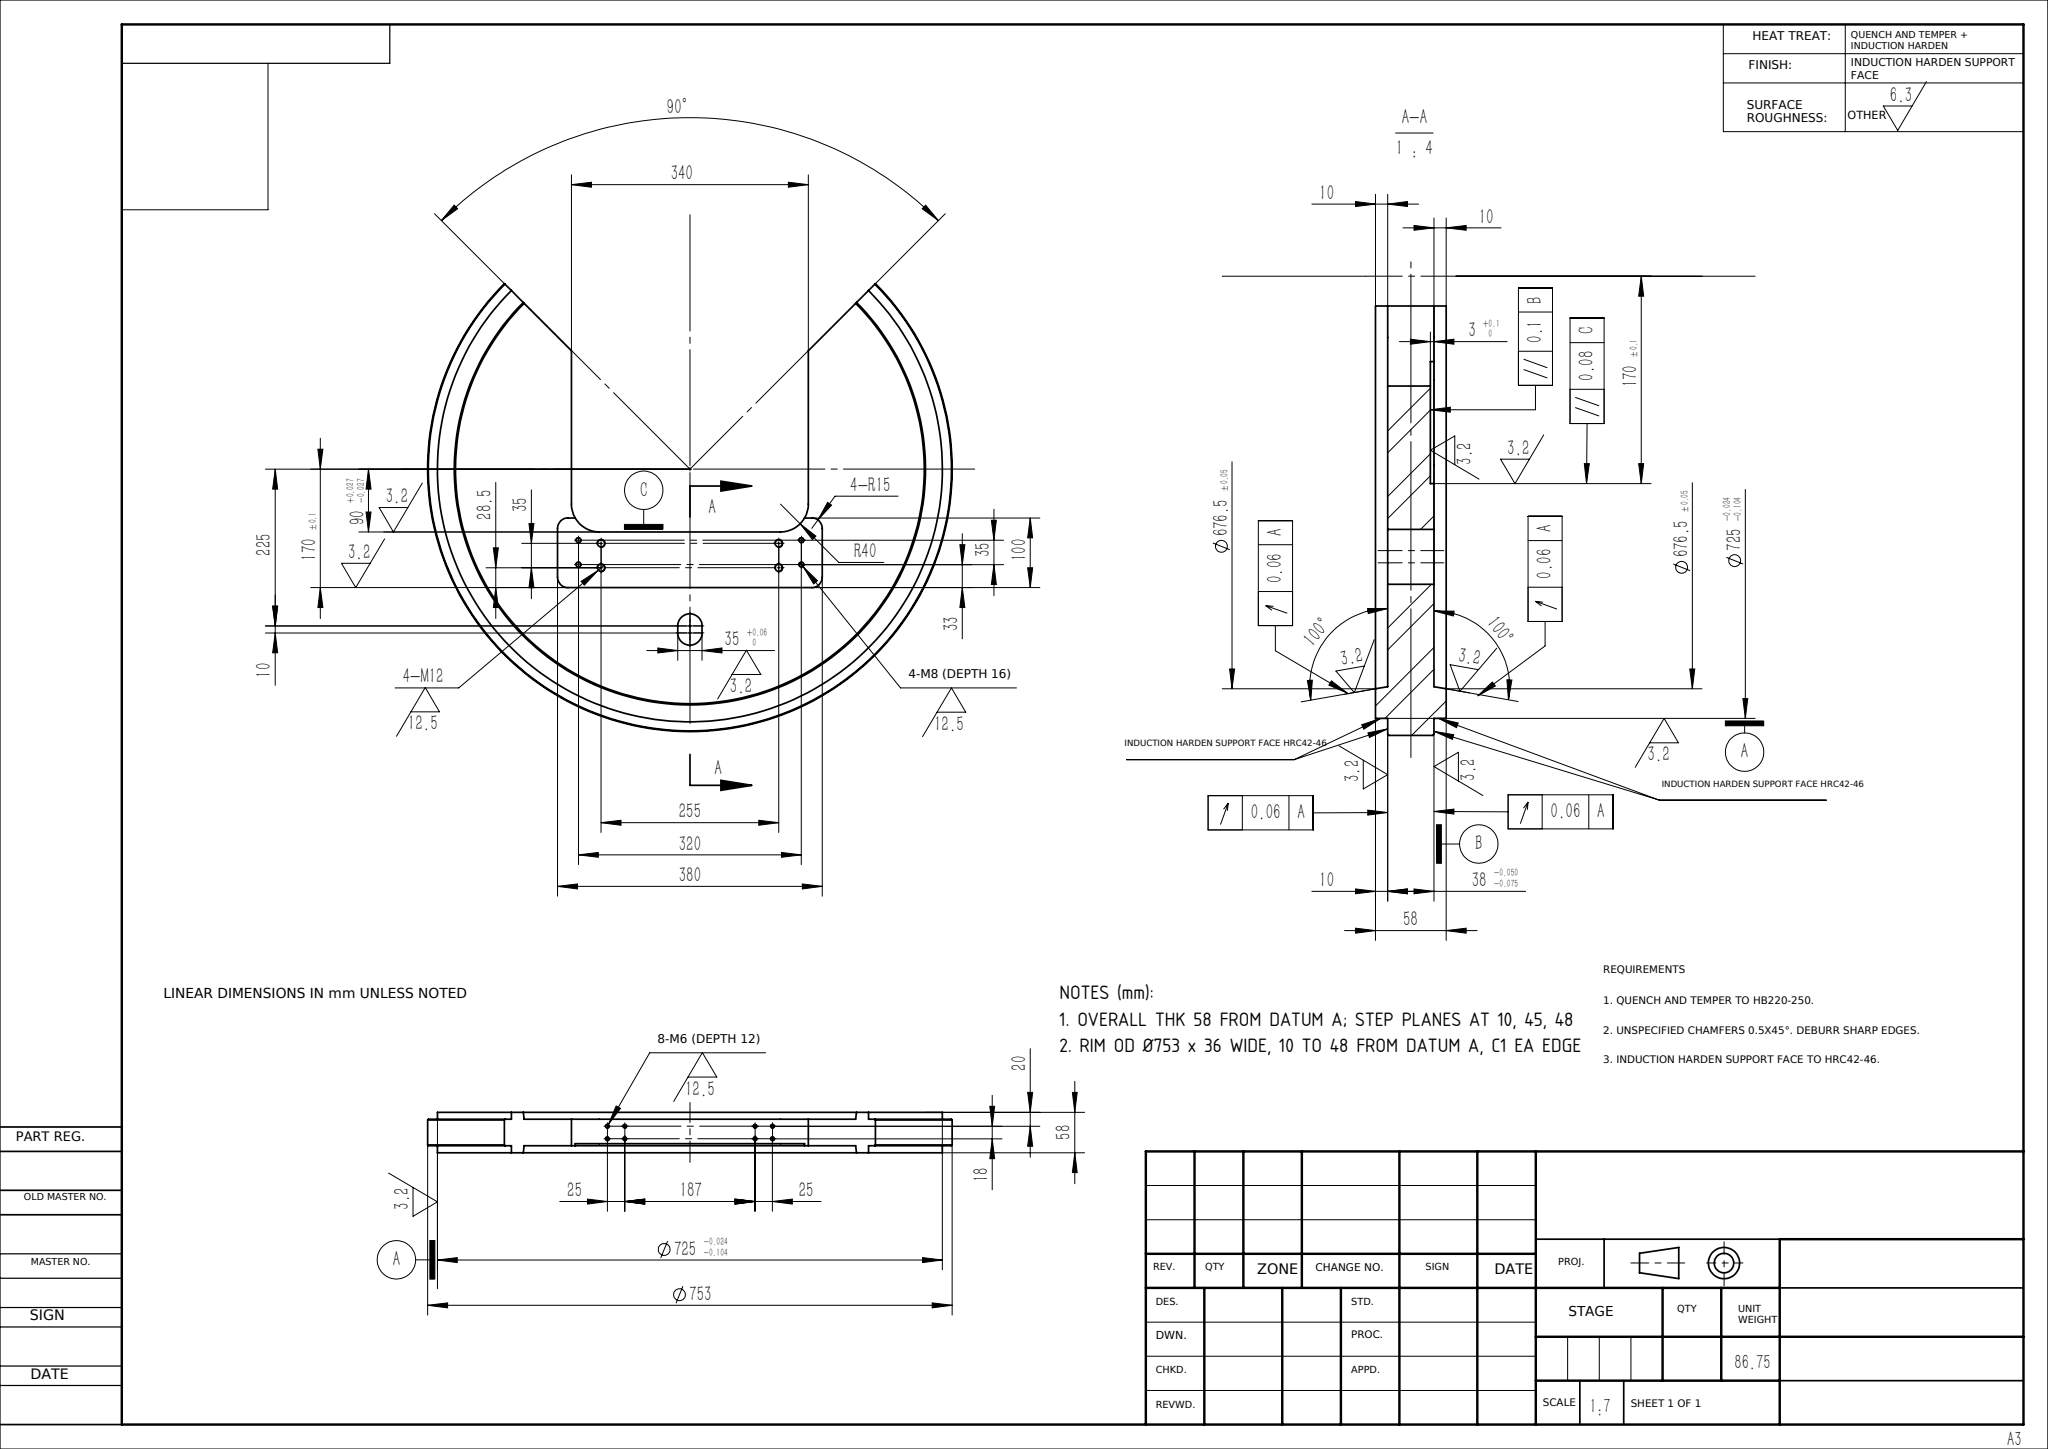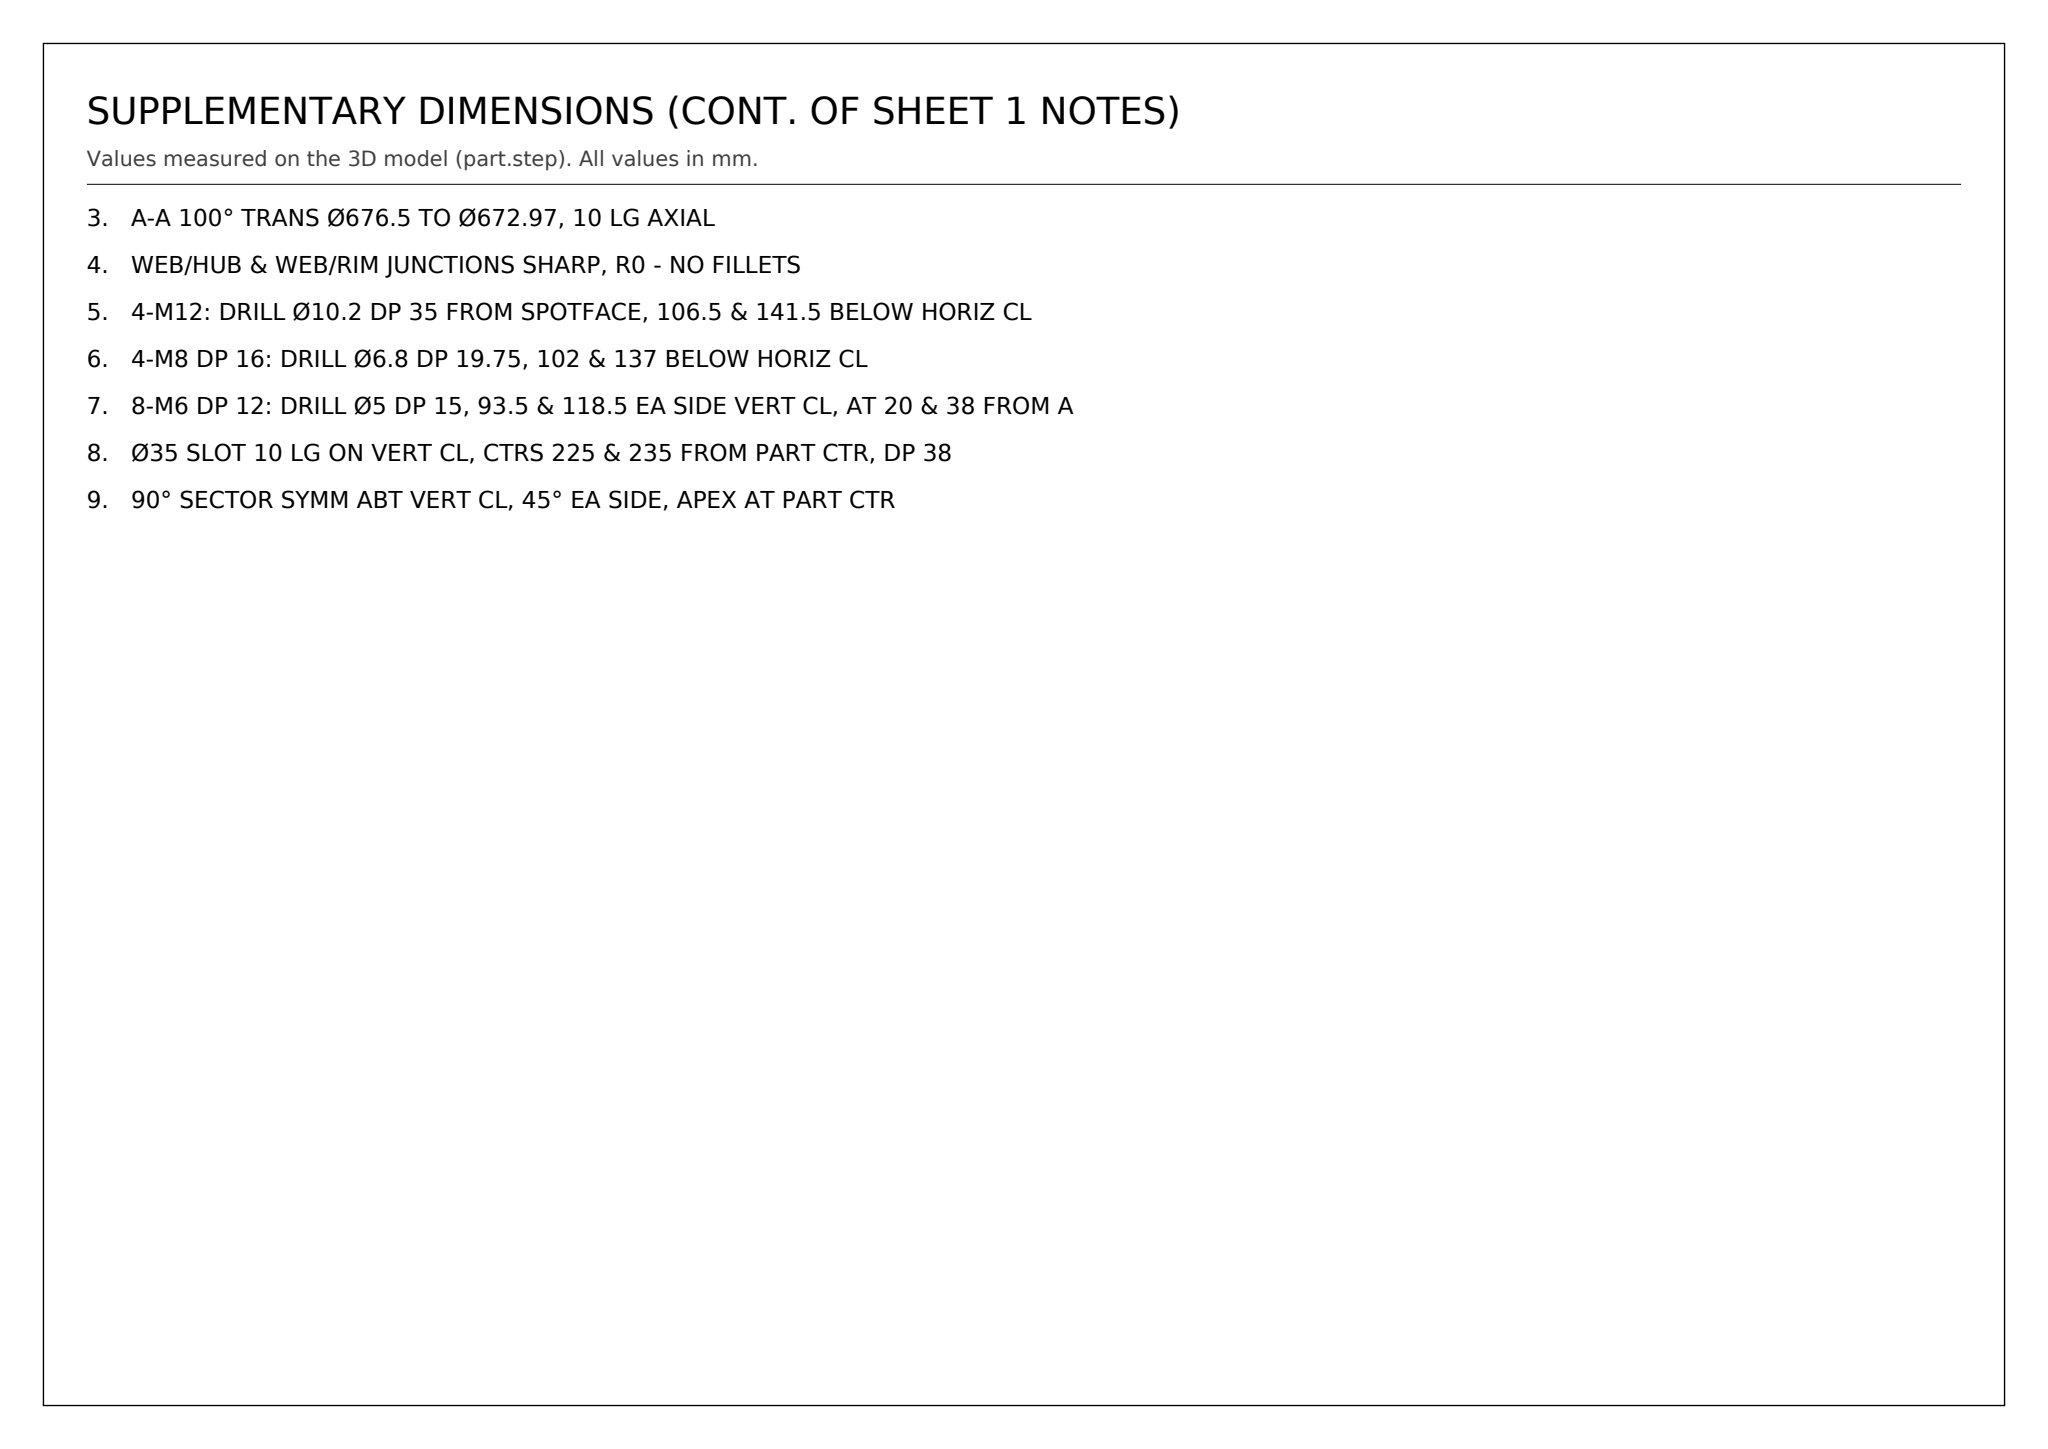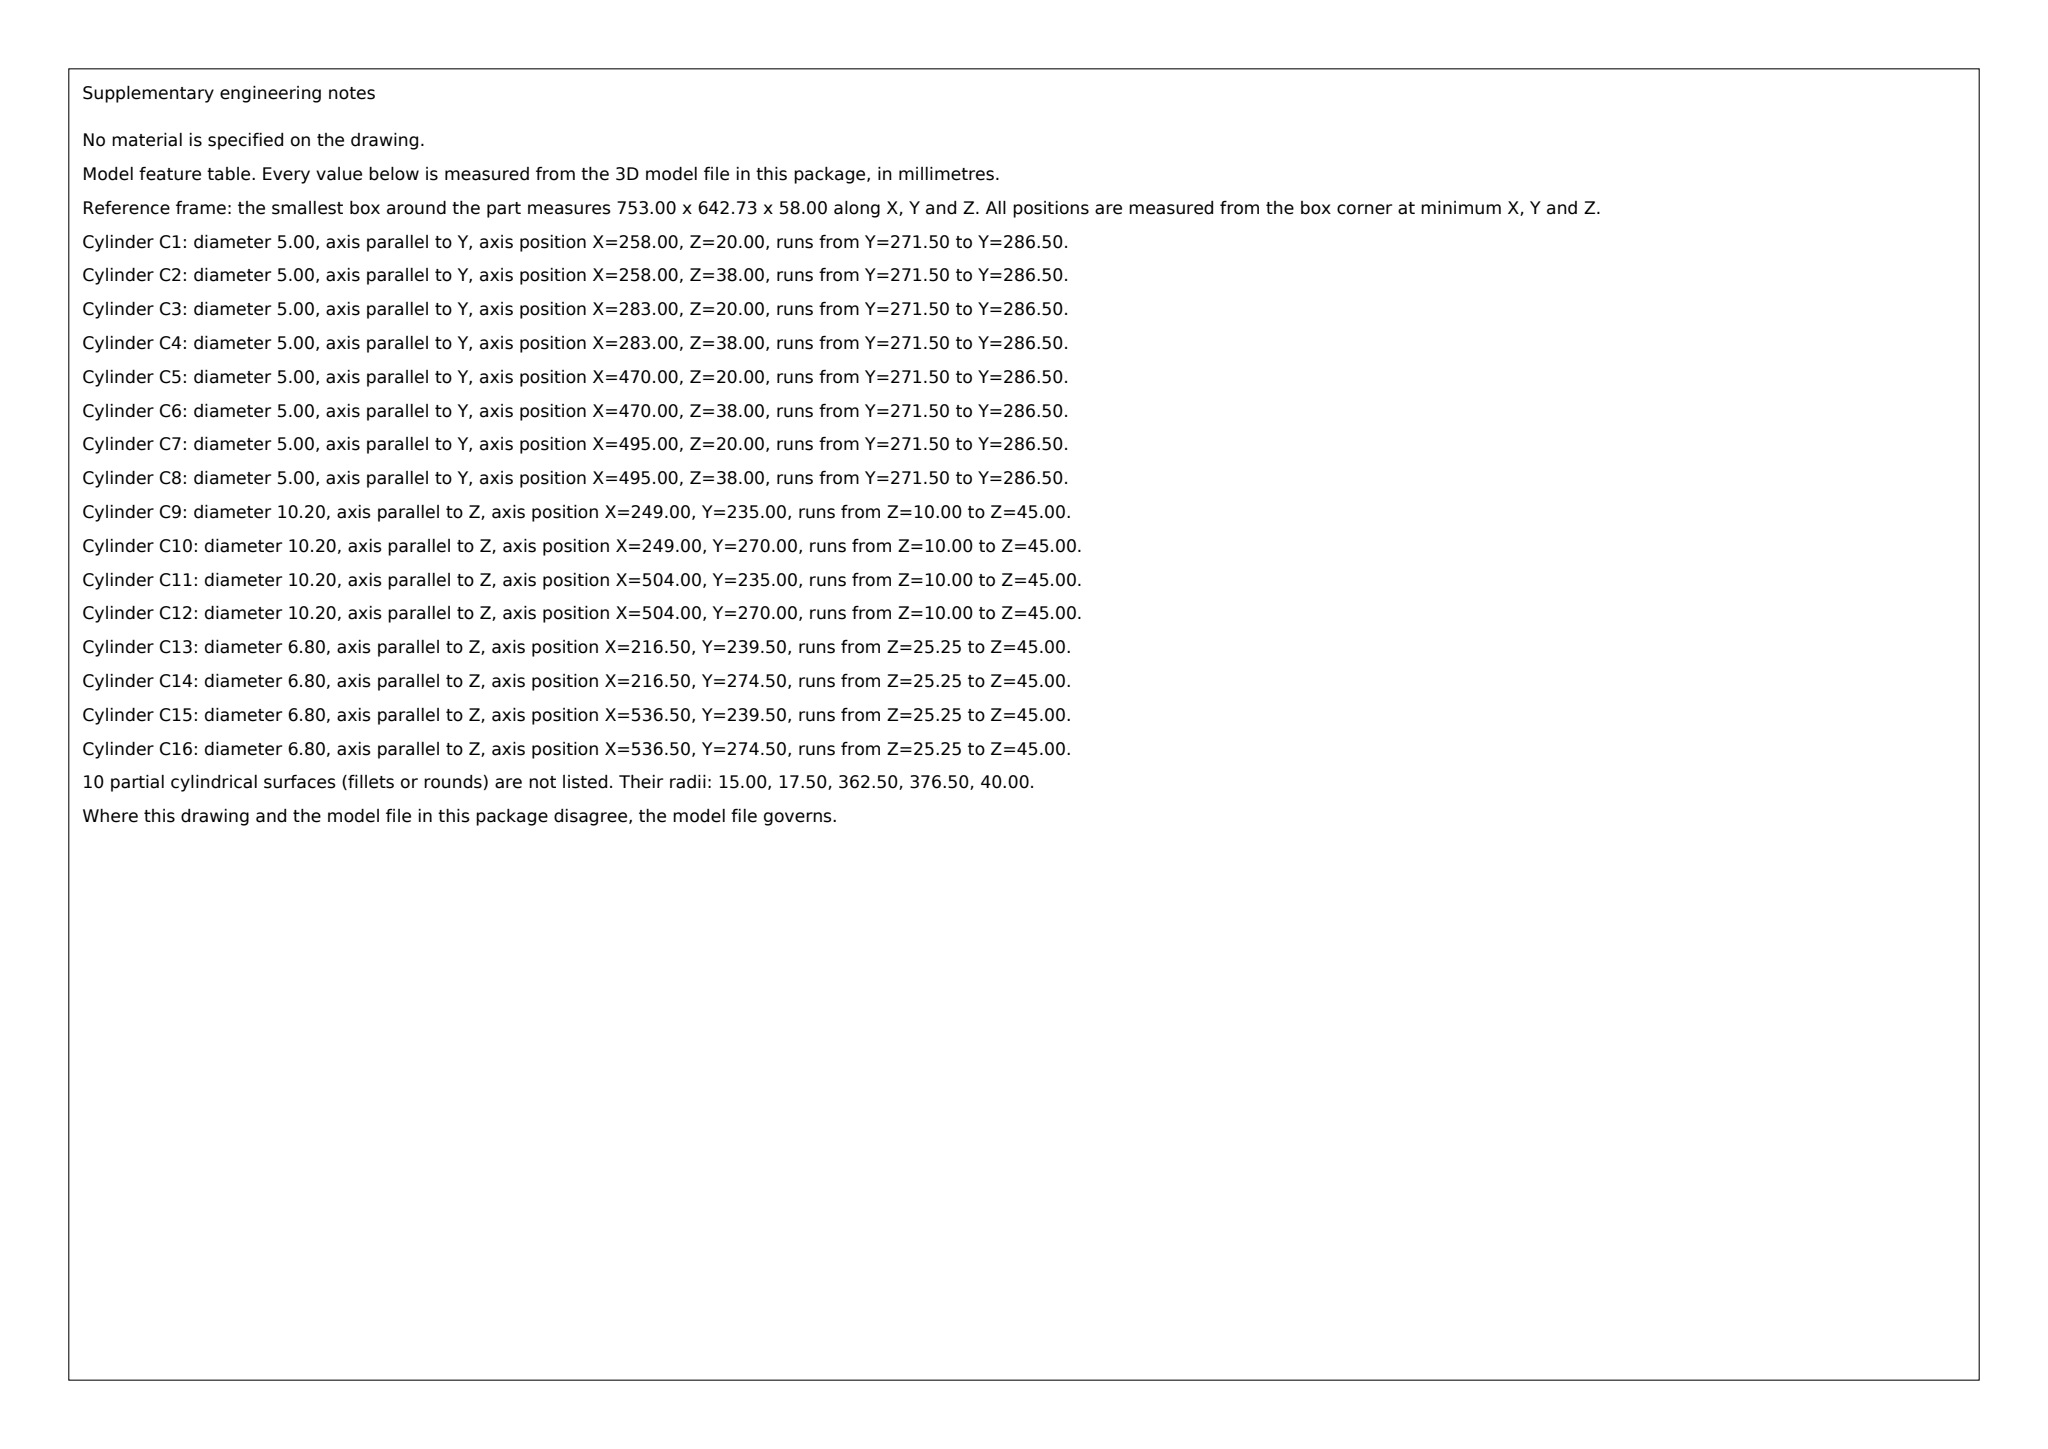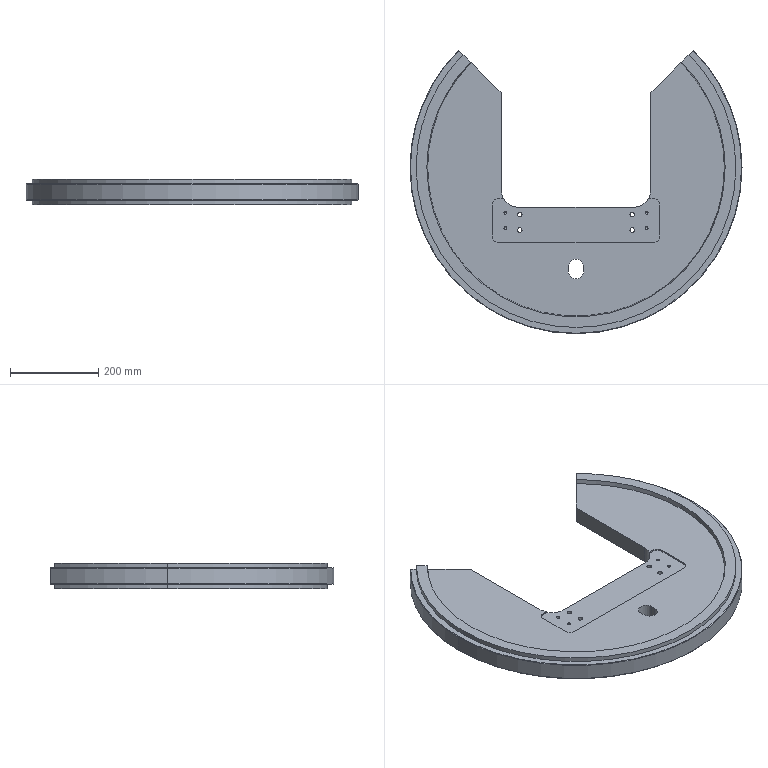Part | SolidWorks | mm | 1 solid | 104 faces | box 753 x 642.73 x 58 mm | volume 11122433 mm3 | cylinder 49 | cone 36 | plane 19 | commonest cylinder face diameters 5 x16 10.2 x8 6.8 x8 725 x6 30 x4 753 x3 80 x2 35 x2
Drawing notes:
OVERALL THK 58 FROM DATUM A; STEP PLANES AT 10, 45, 48 | from the solid: z planes 0,10,45,48,58; bbox z=58
RIM OD Ø753 x 36 WIDE, 10 TO 48 FROM DATUM A, C1 EA EDGE | from the solid: cyl[753 dia, z, len 36]; cones[90°, 753 & 751] = 1x45°; planes z=10, z=48
A-A 100° TRANS Ø676.5 TO Ø672.97, 10 LG AXIAL | from the solid: cones[20.0 incl, ref_dia 676.5] to [20.0, 672.973]; radial drop 1.76 over 10 axial
WEB/HUB & WEB/RIM JUNCTIONS SHARP, R0 - NO FILLETS | from the solid: fillet_radii: [] (no fillet faces in model)
4-M12: DRILL Ø10.2 DP 35 FROM SPOTFACE, 106.5 & 141.5 BELOW HORIZ CL | from the solid: Ø10.2 z-axis cyls L=35 at (249,235)(249,270)(504,235)(504,270), z=45 to 10; CL 376.5
4-M8 DP 16: DRILL Ø6.8 DP 19.75, 102 & 137 BELOW HORIZ CL | from the solid: Ø6.8 cyls axis z len 19.75 at (216.5,239.5)(216.5,274.5)(536.5,239.5)(536.5,274.5); CL 376.5
8-M6 DP 12: DRILL Ø5 DP 15, 93.5 & 118.5 EA SIDE VERT CL, AT 20 & 38 FROM A | from the solid: Ø5 cyls axis y len 15 at x=258,283,470,495 and z=20,38; CL x=376.5
Ø35 SLOT 10 LG ON VERT CL, CTRS 225 & 235 FROM PART CTR, DP 38 | from the solid: two Ø35 z-axis cyls L=38 at (376.5,141.5) & (376.5,151.5); part ctr (376.5,376.5)
90° SECTOR SYMM ABT VERT CL, 45° EA SIDE, APEX AT PART CTR | from the solid: bbox y 642.726 = 376.5+376.5/√2; apex at ctr (376.5,376.5), symm abt Ø35 slot CL
build123d program:
from build123d import *

# Parameters (mm, degrees)
CUT_EXTRUDE1_DEPTH    = 536.601
SKETCH3_W             = 340
SKETCH3_H             = 260
CUT_EXTRUDE2_DEPTH    = 536.601
FILLET1_R             = 40
CUT_EXTRUDE4_DEPTH    = 3
M8_TAPPED_HOLE1_D     = 6.8
M8_TAPPED_HOLE1_DEPTH = 19.75
M8_TAPPED_HOLE1_TIP   = 2.043
M12_TAPPED_HOLE1_D    = 10.2
M6_TAPPED_HOLE1_D     = 5
M6_TAPPED_HOLE1_DEPTH = 15
M6_TAPPED_HOLE1_TIP   = 1.502
CUT_EXTRUDE5_DEPTH    = 535.611
CHAMFER1_SIZE         = 1


with BuildPart() as part:
    # Sketch1 → Revolve1 (revolve)
    with BuildSketch(Plane(origin=(0, 0, 0), x_dir=(1, 0, 0), z_dir=(0, 1, 0))):
        Polygon((376.5, -19), (376.5, 19), (362.5, 19), (362.5, 29), (338.25, 29), (336.487, 19), (0, 19), (0, -19), (336.487, -19), (338.25, -29), (362.5, -29), (362.5, -19), align=None)
    revolve(axis=Axis((0, 0, 0), (0, 0, -1)))

    # Sketch2 → Cut-Extrude1 (cut, through all)
    with BuildSketch(Plane.XY.offset(29)):
        with BuildLine():
            Line((0, 0), (-266.226, 266.226))
            ThreePointArc((-266.226, 266.226), (0, 376.5), (266.226, 266.226))
            Line((266.226, 266.226), (0, 0))
        make_face()
    extrude(amount=-CUT_EXTRUDE1_DEPTH, mode=Mode.SUBTRACT)

    # Sketch3 → Cut-Extrude2 (cut, through all)
    with BuildSketch(Plane.XY.offset(29)):
        with Locations((0, 40)):
            Rectangle(SKETCH3_W, SKETCH3_H)
    extrude(amount=-CUT_EXTRUDE2_DEPTH, mode=Mode.SUBTRACT)

    # Fillet1
    fillet1_edges = [part.edges().sort_by_distance(p)[0] for p in [
        (-170, -90, 0),
        (170, -90, 0),
    ]]
    fillet(fillet1_edges, radius=FILLET1_R)

    # Sketch5 → Cut-Extrude4 (cut)
    with BuildSketch(Plane.XY.offset(19)):
        with BuildLine():
            Line((-175, -170), (175, -170))
            ThreePointArc((175, -170), (185.607, -165.607), (190, -155))
            Line((190, -155), (190, -85))
            ThreePointArc((190, -85), (185.607, -74.393), (175, -70))
            Line((175, -70), (-175, -70))
            ThreePointArc((-175, -70), (-185.607, -74.393), (-190, -85))
            Line((-190, -85), (-190, -155))
            ThreePointArc((-190, -155), (-185.607, -165.607), (-175, -170))
        make_face()
    extrude(amount=-CUT_EXTRUDE4_DEPTH, mode=Mode.SUBTRACT)

    # M8 Tapped Hole1
    with Locations(Plane.XY.offset(16)):
        with Locations((-160, -102), (-160, -137), (160, -102), (160, -137)):
            Hole(M8_TAPPED_HOLE1_D / 2, depth=M8_TAPPED_HOLE1_DEPTH)
            with Locations((0, 0, -(M8_TAPPED_HOLE1_DEPTH + M8_TAPPED_HOLE1_TIP / 2))):  # 118° drill point
                Cone(0, M8_TAPPED_HOLE1_D / 2, M8_TAPPED_HOLE1_TIP, mode=Mode.SUBTRACT)

    # M12 Tapped Hole1 (through all)
    with Locations(Plane.XY.offset(16)):
        with Locations((-127.5, -106.5), (127.5, -106.5), (127.5, -141.5), (-127.5, -141.5)):
            Hole(M12_TAPPED_HOLE1_D / 2)

    # M6 Tapped Hole1
    with Locations(Plane(origin=(0, -90, 0), x_dir=(1, 0, 0), z_dir=(0, 1, 0))):
        with Locations((-118.5, 9), (-118.5, -9), (-93.5, 9), (-93.5, -9), (118.5, -9), (118.5, 9), (93.5, -9), (93.5, 9)):
            Hole(M6_TAPPED_HOLE1_D / 2, depth=M6_TAPPED_HOLE1_DEPTH)
            with Locations((0, 0, -(M6_TAPPED_HOLE1_DEPTH + M6_TAPPED_HOLE1_TIP / 2))):  # 118° drill point
                Cone(0, M6_TAPPED_HOLE1_D / 2, M6_TAPPED_HOLE1_TIP, mode=Mode.SUBTRACT)

    # Sketch13 → Cut-Extrude5 (cut, through all)
    with BuildSketch(Plane(origin=(0, 0, -19), x_dir=(-1, 0, 0), z_dir=(0, 0, -1))):
        with BuildLine():
            Line((-17.5, -235), (-17.5, -225))
            ThreePointArc((-17.5, -225), (0, -207.5), (17.5, -225))
            Line((17.5, -225), (17.5, -235))
            ThreePointArc((17.5, -235), (0, -252.5), (-17.5, -235))
        make_face()
    extrude(amount=-CUT_EXTRUDE5_DEPTH, mode=Mode.SUBTRACT)

    # Chamfer1
    chamfer1_edges = [part.edges().sort_by_distance(p)[0] for p in [
        (0, -376.5, -19),
        (0, -376.5, 19),
    ]]
    chamfer(chamfer1_edges, length=CHAMFER1_SIZE)


solid = part.part